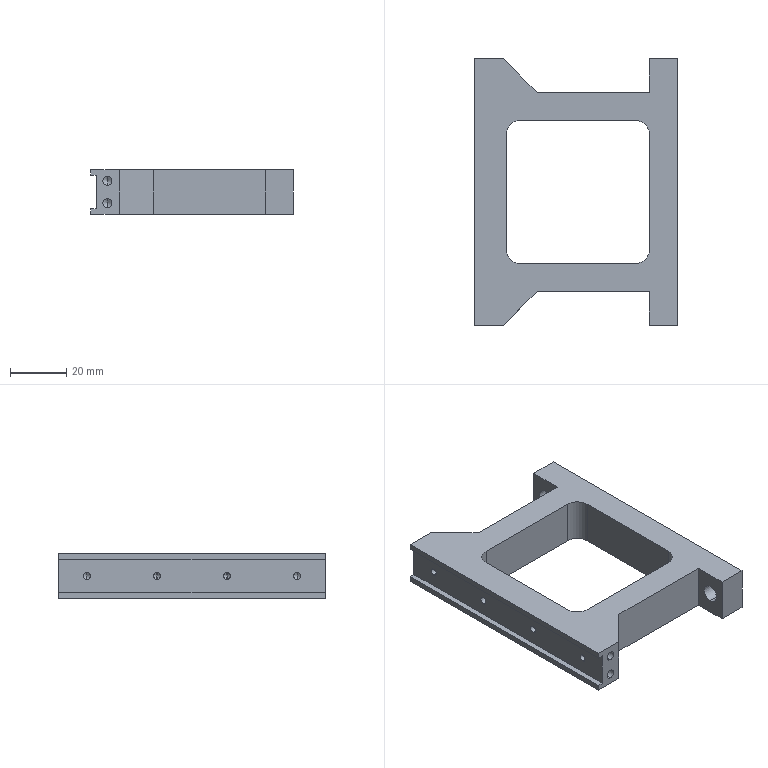Component | SolidWorks | 7.1.02.0001.00.00-0049-1 | 1 solid | 62 faces | box 72.3 x 95 x 16 mm | volume 47605 mm3 | cylinder 24 | plane 22 | cone 16 | commonest cylinder face diameters 3.3 x8 2.5 x8 6 x4 10 x4
build123d program:
from build123d import *

# Parameters (mm, degrees)
SKETCH1_W                           = 51
SKETCH1_H                           = 51
BOSS_EXTRUDE1_DEPTH                 = 16
FILLET1_R                           = 5
SKETCH2_R                           = 3
CUT_EXTRUDE1_DEPTH                  = 10
SKETCH3_W                           = 2
SKETCH3_H                           = 12
CUT_EXTRUDE2_DEPTH                  = 103.897
M3X0_5_TAPPED_HOLE1_D               = 2.5
M3X0_5_TAPPED_HOLE1_DEPTH           = 7.5
M3X0_5_TAPPED_HOLE1_TIP             = 0.7511
M4X0_7_TAPPED_HOLE1_D               = 3.3
M4X0_7_TAPPED_HOLE1_DEPTH           = 10.1
M4X0_7_TAPPED_HOLE1_TIP             = 0.9914
M4X0_7_TAPPED_HOLE1_ON_FACE_2_D     = 3.3
M4X0_7_TAPPED_HOLE1_ON_FACE_2_DEPTH = 10.1
M4X0_7_TAPPED_HOLE1_ON_FACE_2_TIP   = 0.9914


with BuildPart() as part:
    # Sketch1 → Boss-Extrude1 (new body)
    with BuildSketch(Plane.XY):
        Polygon((-25.85, 47.5), (-13.85, 35.5), (26.15, 35.5), (26.15, 47.5), (36.15, 47.5), (36.15, -47.5), (26.15, -47.5), (26.15, -35.5), (-13.85, -35.5), (-25.85, -47.5), (-36.15, -47.5), (-36.15, 47.5), align=None)
        with Locations((0.65, 0)):
            Rectangle(SKETCH1_W, SKETCH1_H, mode=Mode.SUBTRACT)
    extrude(amount=BOSS_EXTRUDE1_DEPTH)

    # Fillet1
    fillet1_edges = [part.edges().sort_by_distance(p)[0] for p in [
        (-24.85, 25.5, 8),
        (-24.85, -25.5, 8),
        (26.15, -25.5, 8),
        (26.15, 25.5, 8),
    ]]
    fillet(fillet1_edges, radius=FILLET1_R)

    # Sketch2 → Cut-Extrude1 (cut)
    with BuildSketch(Plane(origin=(36.15, 0, 0), x_dir=(0, 0, -1), z_dir=(1, 0, 0))):
        with Locations((-8, 41.5)):
            Circle(SKETCH2_R)
        with Locations((-8, -41.5)):
            Circle(SKETCH2_R)
    extrude(amount=-CUT_EXTRUDE1_DEPTH, mode=Mode.SUBTRACT)

    # Sketch3 → Cut-Extrude2 (cut, through all)
    with BuildSketch(Plane.XZ.offset(47.5)):
        with Locations((-35.15, 8)):
            Rectangle(SKETCH3_W, SKETCH3_H)
    extrude(amount=-CUT_EXTRUDE2_DEPTH, mode=Mode.SUBTRACT)

    # M3x0.5 Tapped Hole1
    with Locations(Plane(origin=(-34.15, -37.5, 8), x_dir=(0, 0, -1), z_dir=(-1, 0, 0))):
        with Locations((0, 0), (0, -25), (0, -50), (0, -75)):
            Hole(M3X0_5_TAPPED_HOLE1_D / 2, depth=M3X0_5_TAPPED_HOLE1_DEPTH)
            with Locations((0, 0, -(M3X0_5_TAPPED_HOLE1_DEPTH + M3X0_5_TAPPED_HOLE1_TIP / 2))):  # 118° drill point
                Cone(0, M3X0_5_TAPPED_HOLE1_D / 2, M3X0_5_TAPPED_HOLE1_TIP, mode=Mode.SUBTRACT)

    # M4x0.7 Tapped Hole1
    with Locations(Plane(origin=(-30.15, -47.5, 4), x_dir=(0, 0, -1), z_dir=(0, -1, 0))):
        with Locations((0, 0), (-8, 0)):
            Hole(M4X0_7_TAPPED_HOLE1_D / 2, depth=M4X0_7_TAPPED_HOLE1_DEPTH)
            with Locations((0, 0, -(M4X0_7_TAPPED_HOLE1_DEPTH + M4X0_7_TAPPED_HOLE1_TIP / 2))):  # 118° drill point
                Cone(0, M4X0_7_TAPPED_HOLE1_D / 2, M4X0_7_TAPPED_HOLE1_TIP, mode=Mode.SUBTRACT)

    # M4x0.7 Tapped Hole1 on face 2
    with Locations(Plane(origin=(-30.15, 47.5, 4), x_dir=(0, 0, 1), z_dir=(0, 1, 0))):
        with Locations((0, 0), (8, 0)):
            Hole(M4X0_7_TAPPED_HOLE1_ON_FACE_2_D / 2, depth=M4X0_7_TAPPED_HOLE1_ON_FACE_2_DEPTH)
            with Locations((0, 0, -(M4X0_7_TAPPED_HOLE1_ON_FACE_2_DEPTH + M4X0_7_TAPPED_HOLE1_ON_FACE_2_TIP / 2))):  # 118° drill point
                Cone(0, M4X0_7_TAPPED_HOLE1_ON_FACE_2_D / 2, M4X0_7_TAPPED_HOLE1_ON_FACE_2_TIP, mode=Mode.SUBTRACT)


solid = part.part

# Placed as in the assembly
solid = solid.moved(Location((-0.8138, -1.184, -8), (0, 0, 0)))